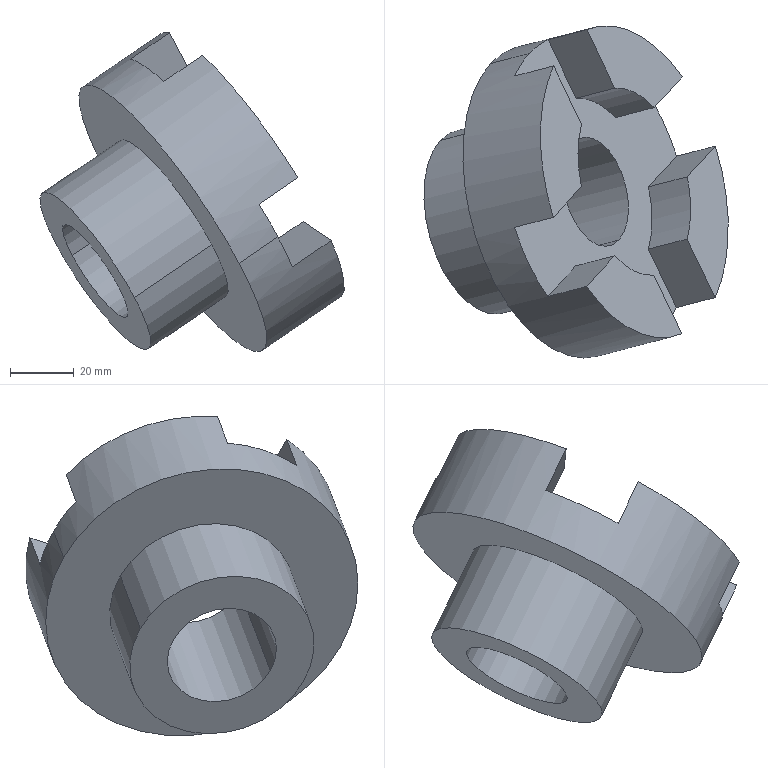Component | SolidWorks | CrusherFrameCoupling-1 | 1 solid | 25 faces | box 95.28 x 104.07 x 100.03 mm | volume 201382 mm3 | plane 15 | cylinder 10 | commonest cylinder face diameters 60 x4 59 x2 100 x2 35 x2
STEP:
#1=COLOUR_RGB('',0.7922,0.8196,0.9333);
#2=FILL_AREA_STYLE_COLOUR('',#1);
#3=FILL_AREA_STYLE('',(#2));
#4=SURFACE_STYLE_FILL_AREA(#3);
#5=SURFACE_SIDE_STYLE('',(#4));
#6=SURFACE_STYLE_USAGE(.BOTH.,#5);
#7=PRESENTATION_STYLE_ASSIGNMENT((#6));
#8=CARTESIAN_POINT('',(13.885,-5.17,1.625));
#9=VERTEX_POINT('',#8);
#10=CARTESIAN_POINT('',(14.849,-7.18,0.9731));
#11=VERTEX_POINT('',#10);
#12=CARTESIAN_POINT('',(14.367,-6.175,1.299));
#13=DIRECTION('',(0.8088,0.2094,0.5495));
#14=DIRECTION('',(-0.4148,0.8655,0.2808));
#15=AXIS2_PLACEMENT_3D('',#12,#13,#14);
#16=CIRCLE('',#15,1.161);
#17=EDGE_CURVE('',#9,#11,#16,.T.);
#18=ORIENTED_EDGE('',*,*,#17,.T.);
#19=CARTESIAN_POINT('',(15.804,-6.933,1.622));
#20=VERTEX_POINT('',#19);
#21=CARTESIAN_POINT('',(16.76,-6.685,2.271));
#22=DIRECTION('',(0.8088,0.2094,0.5495));
#23=VECTOR('',#22,39.37);
#24=LINE('',#21,#23);
#25=EDGE_CURVE('',#11,#20,#24,.T.);
#26=ORIENTED_EDGE('',*,*,#25,.T.);
#27=CARTESIAN_POINT('',(14.841,-4.922,2.274));
#28=VERTEX_POINT('',#27);
#29=CARTESIAN_POINT('',(15.323,-5.927,1.948));
#30=DIRECTION('',(0.8088,0.2094,0.5495));
#31=DIRECTION('',(-0.4148,0.8655,0.2808));
#32=AXIS2_PLACEMENT_3D('',#29,#30,#31);
#33=CIRCLE('',#32,1.161);
#34=EDGE_CURVE('',#28,#20,#33,.T.);
#35=ORIENTED_EDGE('',*,*,#34,.F.);
#36=CARTESIAN_POINT('',(15.796,-4.675,2.923));
#37=DIRECTION('',(0.8088,0.2094,0.5495));
#38=VECTOR('',#37,39.37);
#39=LINE('',#36,#38);
#40=EDGE_CURVE('',#9,#28,#39,.T.);
#41=ORIENTED_EDGE('',*,*,#40,.F.);
#42=EDGE_LOOP('',(#18,#26,#35,#41));
#43=FACE_OUTER_BOUND('',#42,.T.);
#44=CARTESIAN_POINT('',(16.278,-5.68,2.597));
#45=DIRECTION('',(0.8088,0.2094,0.5495));
#46=DIRECTION('',(-0.4148,0.8655,0.2808));
#47=AXIS2_PLACEMENT_3D('',#44,#45,#46);
#48=CYLINDRICAL_SURFACE('',#47,1.161);
#49=ADVANCED_FACE('',(#43),#48,.T.);
#50=CARTESIAN_POINT('',(14.506,-4.224,2.501));
#51=VERTEX_POINT('',#50);
#52=CARTESIAN_POINT('',(16.139,-7.631,1.395));
#53=VERTEX_POINT('',#52);
#54=CARTESIAN_POINT('',(15.323,-5.927,1.948));
#55=DIRECTION('',(0.8088,0.2094,0.5495));
#56=DIRECTION('',(-0.4148,0.8655,0.2808));
#57=AXIS2_PLACEMENT_3D('',#54,#55,#56);
#58=CIRCLE('',#57,1.969);
#59=EDGE_CURVE('',#51,#53,#58,.T.);
#60=ORIENTED_EDGE('',*,*,#59,.T.);
#61=CARTESIAN_POINT('',(16.617,-7.507,1.72));
#62=VERTEX_POINT('',#61);
#63=CARTESIAN_POINT('',(17.095,-7.384,2.044));
#64=DIRECTION('',(0.8088,0.2094,0.5495));
#65=VECTOR('',#64,39.37);
#66=LINE('',#63,#65);
#67=EDGE_CURVE('',#53,#62,#66,.T.);
#68=ORIENTED_EDGE('',*,*,#67,.T.);
#69=CARTESIAN_POINT('',(16.386,-7.677,2.125));
#70=VERTEX_POINT('',#69);
#71=CARTESIAN_POINT('',(15.8,-5.804,2.273));
#72=DIRECTION('',(-0.8088,-0.2094,-0.5495));
#73=DIRECTION('',(-0.4168,-0.4551,0.7869));
#74=AXIS2_PLACEMENT_3D('',#71,#72,#73);
#75=CIRCLE('',#74,1.969);
#76=EDGE_CURVE('',#62,#70,#75,.T.);
#77=ORIENTED_EDGE('',*,*,#76,.T.);
#78=CARTESIAN_POINT('',(16.864,-7.554,2.449));
#79=VERTEX_POINT('',#78);
#80=CARTESIAN_POINT('',(16.864,-7.554,2.449));
#81=DIRECTION('',(0.8088,0.2094,0.5495));
#82=VECTOR('',#81,39.37);
#83=LINE('',#80,#82);
#84=EDGE_CURVE('',#70,#79,#83,.T.);
#85=ORIENTED_EDGE('',*,*,#84,.T.);
#86=CARTESIAN_POINT('',(15.688,-6.973,3.959));
#87=VERTEX_POINT('',#86);
#88=CARTESIAN_POINT('',(16.278,-5.68,2.597));
#89=DIRECTION('',(0.8088,0.2094,0.5495));
#90=DIRECTION('',(-0.4148,0.8655,0.2808));
#91=AXIS2_PLACEMENT_3D('',#88,#89,#90);
#92=CIRCLE('',#91,1.969);
#93=EDGE_CURVE('',#87,#79,#92,.T.);
#94=ORIENTED_EDGE('',*,*,#93,.F.);
#95=CARTESIAN_POINT('',(15.21,-7.097,3.634));
#96=VERTEX_POINT('',#95);
#97=CARTESIAN_POINT('',(15.688,-6.973,3.959));
#98=DIRECTION('',(-0.8088,-0.2094,-0.5495));
#99=VECTOR('',#98,39.37);
#100=LINE('',#97,#99);
#101=EDGE_CURVE('',#87,#96,#100,.T.);
#102=ORIENTED_EDGE('',*,*,#101,.T.);
#103=CARTESIAN_POINT('',(14.802,-6.245,3.911));
#104=VERTEX_POINT('',#103);
#105=CARTESIAN_POINT('',(15.8,-5.804,2.273));
#106=DIRECTION('',(-0.8088,-0.2094,-0.5495));
#107=DIRECTION('',(0.4148,-0.8655,-0.2808));
#108=AXIS2_PLACEMENT_3D('',#105,#106,#107);
#109=CIRCLE('',#108,1.969);
#110=EDGE_CURVE('',#96,#104,#109,.T.);
#111=ORIENTED_EDGE('',*,*,#110,.T.);
#112=CARTESIAN_POINT('',(15.279,-6.122,4.235));
#113=VERTEX_POINT('',#112);
#114=CARTESIAN_POINT('',(15.279,-6.122,4.235));
#115=DIRECTION('',(0.8088,0.2094,0.5495));
#116=VECTOR('',#115,39.37);
#117=LINE('',#114,#116);
#118=EDGE_CURVE('',#104,#113,#117,.T.);
#119=ORIENTED_EDGE('',*,*,#118,.T.);
#120=CARTESIAN_POINT('',(15.282,-4.254,3.52));
#121=VERTEX_POINT('',#120);
#122=CARTESIAN_POINT('',(16.278,-5.68,2.597));
#123=DIRECTION('',(0.8088,0.2094,0.5495));
#124=DIRECTION('',(-0.4148,0.8655,0.2808));
#125=AXIS2_PLACEMENT_3D('',#122,#123,#124);
#126=CIRCLE('',#125,1.969);
#127=EDGE_CURVE('',#121,#113,#126,.T.);
#128=ORIENTED_EDGE('',*,*,#127,.F.);
#129=CARTESIAN_POINT('',(14.804,-4.378,3.195));
#130=VERTEX_POINT('',#129);
#131=CARTESIAN_POINT('',(15.282,-4.254,3.52));
#132=DIRECTION('',(-0.8088,-0.2094,-0.5495));
#133=VECTOR('',#132,39.37);
#134=LINE('',#131,#133);
#135=EDGE_CURVE('',#121,#130,#134,.T.);
#136=ORIENTED_EDGE('',*,*,#135,.T.);
#137=CARTESIAN_POINT('',(14.984,-4.1,2.825));
#138=VERTEX_POINT('',#137);
#139=CARTESIAN_POINT('',(15.8,-5.804,2.273));
#140=DIRECTION('',(-0.8088,-0.2094,-0.5495));
#141=DIRECTION('',(0.4148,-0.8655,-0.2808));
#142=AXIS2_PLACEMENT_3D('',#139,#140,#141);
#143=CIRCLE('',#142,1.969);
#144=EDGE_CURVE('',#130,#138,#143,.T.);
#145=ORIENTED_EDGE('',*,*,#144,.T.);
#146=CARTESIAN_POINT('',(15.461,-3.976,3.15));
#147=DIRECTION('',(0.8088,0.2094,0.5495));
#148=VECTOR('',#147,39.37);
#149=LINE('',#146,#148);
#150=EDGE_CURVE('',#51,#138,#149,.T.);
#151=ORIENTED_EDGE('',*,*,#150,.F.);
#152=EDGE_LOOP('',(#60,#68,#77,#85,#94,#102,#111,#119,#128,#136,#145,#151));
#153=FACE_OUTER_BOUND('',#152,.T.);
#154=CARTESIAN_POINT('',(16.278,-5.68,2.597));
#155=DIRECTION('',(0.8088,0.2094,0.5495));
#156=DIRECTION('',(-0.4148,0.8655,0.2808));
#157=AXIS2_PLACEMENT_3D('',#154,#155,#156);
#158=CYLINDRICAL_SURFACE('',#157,1.969);
#159=ADVANCED_FACE('',(#153),#158,.T.);
#160=CARTESIAN_POINT('',(14.653,-6.771,1.106));
#161=VERTEX_POINT('',#160);
#162=CARTESIAN_POINT('',(14.081,-5.579,1.493));
#163=VERTEX_POINT('',#162);
#164=CARTESIAN_POINT('',(14.367,-6.175,1.299));
#165=DIRECTION('',(0.8088,0.2094,0.5495));
#166=DIRECTION('',(-0.4148,0.8655,0.2808));
#167=AXIS2_PLACEMENT_3D('',#164,#165,#166);
#168=CIRCLE('',#167,0.689);
#169=EDGE_CURVE('',#161,#163,#168,.T.);
#170=ORIENTED_EDGE('',*,*,#169,.F.);
#171=CARTESIAN_POINT('',(16.086,-6.4,2.079));
#172=VERTEX_POINT('',#171);
#173=CARTESIAN_POINT('',(16.564,-6.276,2.404));
#174=DIRECTION('',(0.8088,0.2094,0.5495));
#175=VECTOR('',#174,39.37);
#176=LINE('',#173,#175);
#177=EDGE_CURVE('',#161,#172,#176,.T.);
#178=ORIENTED_EDGE('',*,*,#177,.T.);
#179=CARTESIAN_POINT('',(15.514,-5.207,2.466));
#180=VERTEX_POINT('',#179);
#181=CARTESIAN_POINT('',(15.8,-5.804,2.273));
#182=DIRECTION('',(0.8088,0.2094,0.5495));
#183=DIRECTION('',(-0.4168,-0.4551,0.7869));
#184=AXIS2_PLACEMENT_3D('',#181,#182,#183);
#185=CIRCLE('',#184,0.689);
#186=EDGE_CURVE('',#172,#180,#185,.T.);
#187=ORIENTED_EDGE('',*,*,#186,.T.);
#188=CARTESIAN_POINT('',(15.992,-5.084,2.791));
#189=DIRECTION('',(0.8088,0.2094,0.5495));
#190=VECTOR('',#189,39.37);
#191=LINE('',#188,#190);
#192=EDGE_CURVE('',#163,#180,#191,.T.);
#193=ORIENTED_EDGE('',*,*,#192,.F.);
#194=EDGE_LOOP('',(#170,#178,#187,#193));
#195=FACE_OUTER_BOUND('',#194,.T.);
#196=CARTESIAN_POINT('',(16.278,-5.68,2.597));
#197=DIRECTION('',(0.8088,0.2094,0.5495));
#198=DIRECTION('',(-0.4148,0.8655,0.2808));
#199=AXIS2_PLACEMENT_3D('',#196,#197,#198);
#200=CYLINDRICAL_SURFACE('',#199,0.689);
#201=ADVANCED_FACE('',(#195),#200,.F.);
#202=CARTESIAN_POINT('',(16.93,-5.617,1.614));
#203=VERTEX_POINT('',#202);
#204=CARTESIAN_POINT('',(17.276,-5.239,0.9592));
#205=VERTEX_POINT('',#204);
#206=CARTESIAN_POINT('',(15.662,-7.002,4.008));
#207=DIRECTION('',(0.4168,0.4551,-0.7869));
#208=VECTOR('',#207,39.37);
#209=LINE('',#206,#208);
#210=EDGE_CURVE('',#203,#205,#209,.T.);
#211=ORIENTED_EDGE('',*,*,#210,.F.);
#212=CARTESIAN_POINT('',(16.928,-6.385,1.908));
#213=VERTEX_POINT('',#212);
#214=CARTESIAN_POINT('',(16.278,-5.68,2.597));
#215=DIRECTION('',(0.8088,0.2094,0.5495));
#216=DIRECTION('',(-0.4148,0.8655,0.2808));
#217=AXIS2_PLACEMENT_3D('',#214,#215,#216);
#218=CIRCLE('',#217,1.181);
#219=EDGE_CURVE('',#213,#203,#218,.T.);
#220=ORIENTED_EDGE('',*,*,#219,.F.);
#221=CARTESIAN_POINT('',(17.274,-7.106,1.675));
#222=VERTEX_POINT('',#221);
#223=CARTESIAN_POINT('',(17.3,-7.16,1.657));
#224=DIRECTION('',(-0.4148,0.8655,0.2808));
#225=VECTOR('',#224,39.37);
#226=LINE('',#223,#225);
#227=EDGE_CURVE('',#222,#213,#226,.T.);
#228=ORIENTED_EDGE('',*,*,#227,.F.);
#229=CARTESIAN_POINT('',(16.278,-5.68,2.597));
#230=DIRECTION('',(0.8088,0.2094,0.5495));
#231=DIRECTION('',(-0.4148,0.8655,0.2808));
#232=AXIS2_PLACEMENT_3D('',#229,#230,#231);
#233=CIRCLE('',#232,1.969);
#234=EDGE_CURVE('',#222,#205,#233,.T.);
#235=ORIENTED_EDGE('',*,*,#234,.T.);
#236=EDGE_LOOP('',(#211,#220,#228,#235));
#237=FACE_OUTER_BOUND('',#236,.T.);
#238=CARTESIAN_POINT('',(15.991,-5.994,3.139));
#239=DIRECTION('',(-0.8088,-0.2094,-0.5495));
#240=DIRECTION('',(0.4148,-0.8655,-0.2808));
#241=AXIS2_PLACEMENT_3D('',#238,#239,#240);
#242=PLANE('',#241);
#243=ADVANCED_FACE('',(#237),#242,.F.);
#244=CARTESIAN_POINT('',(16.518,-6.833,2.683));
#245=VERTEX_POINT('',#244);
#246=CARTESIAN_POINT('',(16.889,-7.608,2.432));
#247=DIRECTION('',(-0.4148,0.8655,0.2808));
#248=VECTOR('',#247,39.37);
#249=LINE('',#246,#248);
#250=EDGE_CURVE('',#79,#245,#249,.T.);
#251=ORIENTED_EDGE('',*,*,#250,.T.);
#252=CARTESIAN_POINT('',(16.035,-6.595,3.304));
#253=VERTEX_POINT('',#252);
#254=CARTESIAN_POINT('',(16.278,-5.68,2.597));
#255=DIRECTION('',(0.8088,0.2094,0.5495));
#256=DIRECTION('',(-0.4148,0.8655,0.2808));
#257=AXIS2_PLACEMENT_3D('',#254,#255,#256);
#258=CIRCLE('',#257,1.181);
#259=EDGE_CURVE('',#253,#245,#258,.T.);
#260=ORIENTED_EDGE('',*,*,#259,.F.);
#261=CARTESIAN_POINT('',(15.662,-7.002,4.008));
#262=DIRECTION('',(0.4168,0.4551,-0.7869));
#263=VECTOR('',#262,39.37);
#264=LINE('',#261,#263);
#265=EDGE_CURVE('',#87,#253,#264,.T.);
#266=ORIENTED_EDGE('',*,*,#265,.F.);
#267=ORIENTED_EDGE('',*,*,#93,.T.);
#268=EDGE_LOOP('',(#251,#260,#266,#267));
#269=FACE_OUTER_BOUND('',#268,.T.);
#270=CARTESIAN_POINT('',(15.991,-5.994,3.139));
#271=DIRECTION('',(-0.8088,-0.2094,-0.5495));
#272=DIRECTION('',(0.4148,-0.8655,-0.2808));
#273=AXIS2_PLACEMENT_3D('',#270,#271,#272);
#274=PLANE('',#273);
#275=ADVANCED_FACE('',(#269),#274,.F.);
#276=CARTESIAN_POINT('',(15.626,-5.743,3.58));
#277=VERTEX_POINT('',#276);
#278=CARTESIAN_POINT('',(15.253,-6.15,4.284));
#279=DIRECTION('',(0.4168,0.4551,-0.7869));
#280=VECTOR('',#279,39.37);
#281=LINE('',#278,#280);
#282=EDGE_CURVE('',#113,#277,#281,.T.);
#283=ORIENTED_EDGE('',*,*,#282,.T.);
#284=CARTESIAN_POINT('',(15.627,-4.975,3.286));
#285=VERTEX_POINT('',#284);
#286=CARTESIAN_POINT('',(16.278,-5.68,2.597));
#287=DIRECTION('',(0.8088,0.2094,0.5495));
#288=DIRECTION('',(-0.4148,0.8655,0.2808));
#289=AXIS2_PLACEMENT_3D('',#286,#287,#288);
#290=CIRCLE('',#289,1.181);
#291=EDGE_CURVE('',#285,#277,#290,.T.);
#292=ORIENTED_EDGE('',*,*,#291,.F.);
#293=CARTESIAN_POINT('',(15.256,-4.2,3.537));
#294=DIRECTION('',(0.4148,-0.8655,-0.2808));
#295=VECTOR('',#294,39.37);
#296=LINE('',#293,#295);
#297=EDGE_CURVE('',#121,#285,#296,.T.);
#298=ORIENTED_EDGE('',*,*,#297,.F.);
#299=ORIENTED_EDGE('',*,*,#127,.T.);
#300=EDGE_LOOP('',(#283,#292,#298,#299));
#301=FACE_OUTER_BOUND('',#300,.T.);
#302=CARTESIAN_POINT('',(15.991,-5.994,3.139));
#303=DIRECTION('',(-0.8088,-0.2094,-0.5495));
#304=DIRECTION('',(0.4148,-0.8655,-0.2808));
#305=AXIS2_PLACEMENT_3D('',#302,#303,#304);
#306=PLANE('',#305);
#307=ADVANCED_FACE('',(#301),#306,.F.);
#308=ORIENTED_EDGE('',*,*,#177,.F.);
#309=CARTESIAN_POINT('',(14.367,-6.175,1.299));
#310=DIRECTION('',(0.8088,0.2094,0.5495));
#311=DIRECTION('',(-0.4148,0.8655,0.2808));
#312=AXIS2_PLACEMENT_3D('',#309,#310,#311);
#313=CIRCLE('',#312,0.689);
#314=EDGE_CURVE('',#163,#161,#313,.T.);
#315=ORIENTED_EDGE('',*,*,#314,.F.);
#316=ORIENTED_EDGE('',*,*,#192,.T.);
#317=CARTESIAN_POINT('',(15.8,-5.804,2.273));
#318=DIRECTION('',(0.8088,0.2094,0.5495));
#319=DIRECTION('',(-0.4168,-0.4551,0.7869));
#320=AXIS2_PLACEMENT_3D('',#317,#318,#319);
#321=CIRCLE('',#320,0.689);
#322=EDGE_CURVE('',#180,#172,#321,.T.);
#323=ORIENTED_EDGE('',*,*,#322,.T.);
#324=EDGE_LOOP('',(#308,#315,#316,#323));
#325=FACE_OUTER_BOUND('',#324,.T.);
#326=CARTESIAN_POINT('',(16.278,-5.68,2.597));
#327=DIRECTION('',(0.8088,0.2094,0.5495));
#328=DIRECTION('',(-0.4148,0.8655,0.2808));
#329=AXIS2_PLACEMENT_3D('',#326,#327,#328);
#330=CYLINDRICAL_SURFACE('',#329,0.689);
#331=ADVANCED_FACE('',(#325),#330,.F.);
#332=CARTESIAN_POINT('',(15.692,-3.807,2.745));
#333=VERTEX_POINT('',#332);
#334=CARTESIAN_POINT('',(16.038,-4.527,2.511));
#335=VERTEX_POINT('',#334);
#336=CARTESIAN_POINT('',(15.666,-3.752,2.763));
#337=DIRECTION('',(0.4148,-0.8655,-0.2808));
#338=VECTOR('',#337,39.37);
#339=LINE('',#336,#338);
#340=EDGE_CURVE('',#333,#335,#339,.T.);
#341=ORIENTED_EDGE('',*,*,#340,.T.);
#342=CARTESIAN_POINT('',(16.521,-4.766,1.891));
#343=VERTEX_POINT('',#342);
#344=CARTESIAN_POINT('',(16.278,-5.68,2.597));
#345=DIRECTION('',(0.8088,0.2094,0.5495));
#346=DIRECTION('',(-0.4148,0.8655,0.2808));
#347=AXIS2_PLACEMENT_3D('',#344,#345,#346);
#348=CIRCLE('',#347,1.181);
#349=EDGE_CURVE('',#343,#335,#348,.T.);
#350=ORIENTED_EDGE('',*,*,#349,.F.);
#351=CARTESIAN_POINT('',(16.868,-4.387,1.236));
#352=VERTEX_POINT('',#351);
#353=CARTESIAN_POINT('',(16.894,-4.358,1.186));
#354=DIRECTION('',(-0.4168,-0.4551,0.7869));
#355=VECTOR('',#354,39.37);
#356=LINE('',#353,#355);
#357=EDGE_CURVE('',#352,#343,#356,.T.);
#358=ORIENTED_EDGE('',*,*,#357,.F.);
#359=CARTESIAN_POINT('',(16.278,-5.68,2.597));
#360=DIRECTION('',(0.8088,0.2094,0.5495));
#361=DIRECTION('',(-0.4148,0.8655,0.2808));
#362=AXIS2_PLACEMENT_3D('',#359,#360,#361);
#363=CIRCLE('',#362,1.969);
#364=EDGE_CURVE('',#352,#333,#363,.T.);
#365=ORIENTED_EDGE('',*,*,#364,.T.);
#366=EDGE_LOOP('',(#341,#350,#358,#365));
#367=FACE_OUTER_BOUND('',#366,.T.);
#368=CARTESIAN_POINT('',(15.991,-5.994,3.139));
#369=DIRECTION('',(-0.8088,-0.2094,-0.5495));
#370=DIRECTION('',(0.4148,-0.8655,-0.2808));
#371=AXIS2_PLACEMENT_3D('',#368,#369,#370);
#372=PLANE('',#371);
#373=ADVANCED_FACE('',(#367),#372,.F.);
#374=ORIENTED_EDGE('',*,*,#67,.F.);
#375=CARTESIAN_POINT('',(15.323,-5.927,1.948));
#376=DIRECTION('',(0.8088,0.2094,0.5495));
#377=DIRECTION('',(-0.4148,0.8655,0.2808));
#378=AXIS2_PLACEMENT_3D('',#375,#376,#377);
#379=CIRCLE('',#378,1.969);
#380=EDGE_CURVE('',#53,#51,#379,.T.);
#381=ORIENTED_EDGE('',*,*,#380,.T.);
#382=ORIENTED_EDGE('',*,*,#150,.T.);
#383=CARTESIAN_POINT('',(15.215,-3.93,2.421));
#384=VERTEX_POINT('',#383);
#385=CARTESIAN_POINT('',(15.8,-5.804,2.273));
#386=DIRECTION('',(-0.8088,-0.2094,-0.5495));
#387=DIRECTION('',(0.4148,-0.8655,-0.2808));
#388=AXIS2_PLACEMENT_3D('',#385,#386,#387);
#389=CIRCLE('',#388,1.969);
#390=EDGE_CURVE('',#138,#384,#389,.T.);
#391=ORIENTED_EDGE('',*,*,#390,.T.);
#392=CARTESIAN_POINT('',(15.692,-3.807,2.745));
#393=DIRECTION('',(0.8088,0.2094,0.5495));
#394=VECTOR('',#393,39.37);
#395=LINE('',#392,#394);
#396=EDGE_CURVE('',#384,#333,#395,.T.);
#397=ORIENTED_EDGE('',*,*,#396,.T.);
#398=ORIENTED_EDGE('',*,*,#364,.F.);
#399=CARTESIAN_POINT('',(16.39,-4.51,0.9111));
#400=VERTEX_POINT('',#399);
#401=CARTESIAN_POINT('',(16.868,-4.387,1.236));
#402=DIRECTION('',(-0.8088,-0.2094,-0.5495));
#403=VECTOR('',#402,39.37);
#404=LINE('',#401,#403);
#405=EDGE_CURVE('',#352,#400,#404,.T.);
#406=ORIENTED_EDGE('',*,*,#405,.T.);
#407=CARTESIAN_POINT('',(16.799,-5.362,0.6347));
#408=VERTEX_POINT('',#407);
#409=CARTESIAN_POINT('',(15.8,-5.804,2.273));
#410=DIRECTION('',(-0.8088,-0.2094,-0.5495));
#411=DIRECTION('',(0.4148,-0.8655,-0.2808));
#412=AXIS2_PLACEMENT_3D('',#409,#410,#411);
#413=CIRCLE('',#412,1.969);
#414=EDGE_CURVE('',#400,#408,#413,.T.);
#415=ORIENTED_EDGE('',*,*,#414,.T.);
#416=CARTESIAN_POINT('',(17.276,-5.239,0.9592));
#417=DIRECTION('',(0.8088,0.2094,0.5495));
#418=VECTOR('',#417,39.37);
#419=LINE('',#416,#418);
#420=EDGE_CURVE('',#408,#205,#419,.T.);
#421=ORIENTED_EDGE('',*,*,#420,.T.);
#422=ORIENTED_EDGE('',*,*,#234,.F.);
#423=CARTESIAN_POINT('',(16.796,-7.229,1.35));
#424=VERTEX_POINT('',#423);
#425=CARTESIAN_POINT('',(17.274,-7.106,1.675));
#426=DIRECTION('',(-0.8088,-0.2094,-0.5495));
#427=VECTOR('',#426,39.37);
#428=LINE('',#425,#427);
#429=EDGE_CURVE('',#222,#424,#428,.T.);
#430=ORIENTED_EDGE('',*,*,#429,.T.);
#431=CARTESIAN_POINT('',(15.8,-5.804,2.273));
#432=DIRECTION('',(-0.8088,-0.2094,-0.5495));
#433=DIRECTION('',(-0.4168,-0.4551,0.7869));
#434=AXIS2_PLACEMENT_3D('',#431,#432,#433);
#435=CIRCLE('',#434,1.969);
#436=EDGE_CURVE('',#424,#62,#435,.T.);
#437=ORIENTED_EDGE('',*,*,#436,.T.);
#438=EDGE_LOOP('',(#374,#381,#382,#391,#397,#398,#406,#415,#421,#422,#430,#437));
#439=FACE_OUTER_BOUND('',#438,.T.);
#440=CARTESIAN_POINT('',(16.278,-5.68,2.597));
#441=DIRECTION('',(0.8088,0.2094,0.5495));
#442=DIRECTION('',(-0.4148,0.8655,0.2808));
#443=AXIS2_PLACEMENT_3D('',#440,#441,#442);
#444=CYLINDRICAL_SURFACE('',#443,1.969);
#445=ADVANCED_FACE('',(#439),#444,.T.);
#446=ORIENTED_EDGE('',*,*,#59,.F.);
#447=ORIENTED_EDGE('',*,*,#380,.F.);
#448=EDGE_LOOP('',(#446,#447));
#449=FACE_OUTER_BOUND('',#448,.T.);
#450=ORIENTED_EDGE('',*,*,#34,.T.);
#451=CARTESIAN_POINT('',(15.323,-5.927,1.948));
#452=DIRECTION('',(0.8088,0.2094,0.5495));
#453=DIRECTION('',(-0.4148,0.8655,0.2808));
#454=AXIS2_PLACEMENT_3D('',#451,#452,#453);
#455=CIRCLE('',#454,1.161);
#456=EDGE_CURVE('',#20,#28,#455,.T.);
#457=ORIENTED_EDGE('',*,*,#456,.T.);
#458=EDGE_LOOP('',(#450,#457));
#459=FACE_BOUND('',#458,.T.);
#460=CARTESIAN_POINT('',(14.502,-6.823,3.497));
#461=DIRECTION('',(0.8088,0.2094,0.5495));
#462=DIRECTION('',(-0.4148,0.8655,0.2808));
#463=AXIS2_PLACEMENT_3D('',#460,#461,#462);
#464=PLANE('',#463);
#465=ADVANCED_FACE('',(#449,#459),#464,.F.);
#466=ORIENTED_EDGE('',*,*,#25,.F.);
#467=CARTESIAN_POINT('',(14.367,-6.175,1.299));
#468=DIRECTION('',(0.8088,0.2094,0.5495));
#469=DIRECTION('',(-0.4148,0.8655,0.2808));
#470=AXIS2_PLACEMENT_3D('',#467,#468,#469);
#471=CIRCLE('',#470,1.161);
#472=EDGE_CURVE('',#11,#9,#471,.T.);
#473=ORIENTED_EDGE('',*,*,#472,.T.);
#474=ORIENTED_EDGE('',*,*,#40,.T.);
#475=ORIENTED_EDGE('',*,*,#456,.F.);
#476=EDGE_LOOP('',(#466,#473,#474,#475));
#477=FACE_OUTER_BOUND('',#476,.T.);
#478=CARTESIAN_POINT('',(16.278,-5.68,2.597));
#479=DIRECTION('',(0.8088,0.2094,0.5495));
#480=DIRECTION('',(-0.4148,0.8655,0.2808));
#481=AXIS2_PLACEMENT_3D('',#478,#479,#480);
#482=CYLINDRICAL_SURFACE('',#481,1.161);
#483=ADVANCED_FACE('',(#477),#482,.T.);
#484=ORIENTED_EDGE('',*,*,#17,.F.);
#485=ORIENTED_EDGE('',*,*,#472,.F.);
#486=EDGE_LOOP('',(#484,#485));
#487=FACE_OUTER_BOUND('',#486,.T.);
#488=ORIENTED_EDGE('',*,*,#314,.T.);
#489=ORIENTED_EDGE('',*,*,#169,.T.);
#490=EDGE_LOOP('',(#488,#489));
#491=FACE_BOUND('',#490,.T.);
#492=CARTESIAN_POINT('',(13.883,-6.703,2.213));
#493=DIRECTION('',(0.8088,0.2094,0.5495));
#494=DIRECTION('',(-0.4148,0.8655,0.2808));
#495=AXIS2_PLACEMENT_3D('',#492,#493,#494);
#496=PLANE('',#495);
#497=ADVANCED_FACE('',(#487,#491),#496,.F.);
#498=CARTESIAN_POINT('',(16.041,-6.957,2.358));
#499=VERTEX_POINT('',#498);
#500=CARTESIAN_POINT('',(16.412,-7.731,2.107));
#501=DIRECTION('',(-0.4148,0.8655,0.2808));
#502=VECTOR('',#501,39.37);
#503=LINE('',#500,#502);
#504=EDGE_CURVE('',#70,#499,#503,.T.);
#505=ORIENTED_EDGE('',*,*,#504,.T.);
#506=CARTESIAN_POINT('',(16.041,-6.957,2.358));
#507=DIRECTION('',(0.8088,0.2094,0.5495));
#508=VECTOR('',#507,39.37);
#509=LINE('',#506,#508);
#510=EDGE_CURVE('',#499,#245,#509,.T.);
#511=ORIENTED_EDGE('',*,*,#510,.T.);
#512=ORIENTED_EDGE('',*,*,#250,.F.);
#513=ORIENTED_EDGE('',*,*,#84,.F.);
#514=EDGE_LOOP('',(#505,#511,#512,#513));
#515=FACE_OUTER_BOUND('',#514,.T.);
#516=CARTESIAN_POINT('',(16.889,-7.608,2.432));
#517=DIRECTION('',(-0.4168,-0.4551,0.7869));
#518=DIRECTION('',(-0.4148,0.8655,0.2808));
#519=AXIS2_PLACEMENT_3D('',#516,#517,#518);
#520=PLANE('',#519);
#521=ADVANCED_FACE('',(#515),#520,.F.);
#522=CARTESIAN_POINT('',(15.557,-6.718,2.979));
#523=VERTEX_POINT('',#522);
#524=CARTESIAN_POINT('',(15.184,-7.126,3.684));
#525=DIRECTION('',(0.4168,0.4551,-0.7869));
#526=VECTOR('',#525,39.37);
#527=LINE('',#524,#526);
#528=EDGE_CURVE('',#96,#523,#527,.T.);
#529=ORIENTED_EDGE('',*,*,#528,.T.);
#530=CARTESIAN_POINT('',(15.8,-5.804,2.273));
#531=DIRECTION('',(0.8088,0.2094,0.5495));
#532=DIRECTION('',(-0.4148,0.8655,0.2808));
#533=AXIS2_PLACEMENT_3D('',#530,#531,#532);
#534=CIRCLE('',#533,1.181);
#535=EDGE_CURVE('',#523,#499,#534,.T.);
#536=ORIENTED_EDGE('',*,*,#535,.T.);
#537=ORIENTED_EDGE('',*,*,#504,.F.);
#538=ORIENTED_EDGE('',*,*,#76,.F.);
#539=ORIENTED_EDGE('',*,*,#436,.F.);
#540=CARTESIAN_POINT('',(16.451,-6.509,1.584));
#541=VERTEX_POINT('',#540);
#542=CARTESIAN_POINT('',(16.822,-7.284,1.333));
#543=DIRECTION('',(-0.4148,0.8655,0.2808));
#544=VECTOR('',#543,39.37);
#545=LINE('',#542,#544);
#546=EDGE_CURVE('',#424,#541,#545,.T.);
#547=ORIENTED_EDGE('',*,*,#546,.T.);
#548=CARTESIAN_POINT('',(16.452,-5.741,1.29));
#549=VERTEX_POINT('',#548);
#550=CARTESIAN_POINT('',(15.8,-5.804,2.273));
#551=DIRECTION('',(0.8088,0.2094,0.5495));
#552=DIRECTION('',(-0.4148,0.8655,0.2808));
#553=AXIS2_PLACEMENT_3D('',#550,#551,#552);
#554=CIRCLE('',#553,1.181);
#555=EDGE_CURVE('',#541,#549,#554,.T.);
#556=ORIENTED_EDGE('',*,*,#555,.T.);
#557=CARTESIAN_POINT('',(15.184,-7.126,3.684));
#558=DIRECTION('',(0.4168,0.4551,-0.7869));
#559=VECTOR('',#558,39.37);
#560=LINE('',#557,#559);
#561=EDGE_CURVE('',#549,#408,#560,.T.);
#562=ORIENTED_EDGE('',*,*,#561,.T.);
#563=ORIENTED_EDGE('',*,*,#414,.F.);
#564=CARTESIAN_POINT('',(16.044,-4.889,1.566));
#565=VERTEX_POINT('',#564);
#566=CARTESIAN_POINT('',(16.417,-4.482,0.8619));
#567=DIRECTION('',(-0.4168,-0.4551,0.7869));
#568=VECTOR('',#567,39.37);
#569=LINE('',#566,#568);
#570=EDGE_CURVE('',#400,#565,#569,.T.);
#571=ORIENTED_EDGE('',*,*,#570,.T.);
#572=CARTESIAN_POINT('',(15.56,-4.651,2.187));
#573=VERTEX_POINT('',#572);
#574=CARTESIAN_POINT('',(15.8,-5.804,2.273));
#575=DIRECTION('',(0.8088,0.2094,0.5495));
#576=DIRECTION('',(-0.4148,0.8655,0.2808));
#577=AXIS2_PLACEMENT_3D('',#574,#575,#576);
#578=CIRCLE('',#577,1.181);
#579=EDGE_CURVE('',#565,#573,#578,.T.);
#580=ORIENTED_EDGE('',*,*,#579,.T.);
#581=CARTESIAN_POINT('',(15.189,-3.876,2.438));
#582=DIRECTION('',(0.4148,-0.8655,-0.2808));
#583=VECTOR('',#582,39.37);
#584=LINE('',#581,#583);
#585=EDGE_CURVE('',#384,#573,#584,.T.);
#586=ORIENTED_EDGE('',*,*,#585,.F.);
#587=ORIENTED_EDGE('',*,*,#390,.F.);
#588=ORIENTED_EDGE('',*,*,#144,.F.);
#589=CARTESIAN_POINT('',(15.15,-5.098,2.961));
#590=VERTEX_POINT('',#589);
#591=CARTESIAN_POINT('',(14.779,-4.324,3.213));
#592=DIRECTION('',(0.4148,-0.8655,-0.2808));
#593=VECTOR('',#592,39.37);
#594=LINE('',#591,#593);
#595=EDGE_CURVE('',#130,#590,#594,.T.);
#596=ORIENTED_EDGE('',*,*,#595,.T.);
#597=CARTESIAN_POINT('',(15.149,-5.866,3.256));
#598=VERTEX_POINT('',#597);
#599=CARTESIAN_POINT('',(15.8,-5.804,2.273));
#600=DIRECTION('',(0.8088,0.2094,0.5495));
#601=DIRECTION('',(-0.4148,0.8655,0.2808));
#602=AXIS2_PLACEMENT_3D('',#599,#600,#601);
#603=CIRCLE('',#602,1.181);
#604=EDGE_CURVE('',#590,#598,#603,.T.);
#605=ORIENTED_EDGE('',*,*,#604,.T.);
#606=CARTESIAN_POINT('',(14.776,-6.274,3.96));
#607=DIRECTION('',(0.4168,0.4551,-0.7869));
#608=VECTOR('',#607,39.37);
#609=LINE('',#606,#608);
#610=EDGE_CURVE('',#104,#598,#609,.T.);
#611=ORIENTED_EDGE('',*,*,#610,.F.);
#612=ORIENTED_EDGE('',*,*,#110,.F.);
#613=EDGE_LOOP('',(#529,#536,#537,#538,#539,#547,#556,#562,#563,#571,#580,#586,#587,#588,#596,#605,#611,#612));
#614=FACE_OUTER_BOUND('',#613,.T.);
#615=ORIENTED_EDGE('',*,*,#322,.F.);
#616=ORIENTED_EDGE('',*,*,#186,.F.);
#617=EDGE_LOOP('',(#615,#616));
#618=FACE_BOUND('',#617,.T.);
#619=CARTESIAN_POINT('',(16.412,-7.731,2.107));
#620=DIRECTION('',(-0.8088,-0.2094,-0.5495));
#621=DIRECTION('',(-0.4168,-0.4551,0.7869));
#622=AXIS2_PLACEMENT_3D('',#619,#620,#621);
#623=PLANE('',#622);
#624=ADVANCED_FACE('',(#614,#618),#623,.F.);
#625=ORIENTED_EDGE('',*,*,#227,.T.);
#626=CARTESIAN_POINT('',(16.451,-6.509,1.584));
#627=DIRECTION('',(-0.8088,-0.2094,-0.5495));
#628=VECTOR('',#627,39.37);
#629=LINE('',#626,#628);
#630=EDGE_CURVE('',#213,#541,#629,.T.);
#631=ORIENTED_EDGE('',*,*,#630,.T.);
#632=ORIENTED_EDGE('',*,*,#546,.F.);
#633=ORIENTED_EDGE('',*,*,#429,.F.);
#634=EDGE_LOOP('',(#625,#631,#632,#633));
#635=FACE_OUTER_BOUND('',#634,.T.);
#636=CARTESIAN_POINT('',(17.3,-7.16,1.657));
#637=DIRECTION('',(0.4168,0.4551,-0.7869));
#638=DIRECTION('',(0.4148,-0.8655,-0.2808));
#639=AXIS2_PLACEMENT_3D('',#636,#637,#638);
#640=PLANE('',#639);
#641=ADVANCED_FACE('',(#635),#640,.F.);
#642=ORIENTED_EDGE('',*,*,#610,.T.);
#643=CARTESIAN_POINT('',(15.149,-5.866,3.256));
#644=DIRECTION('',(0.8088,0.2094,0.5495));
#645=VECTOR('',#644,39.37);
#646=LINE('',#643,#645);
#647=EDGE_CURVE('',#598,#277,#646,.T.);
#648=ORIENTED_EDGE('',*,*,#647,.T.);
#649=ORIENTED_EDGE('',*,*,#282,.F.);
#650=ORIENTED_EDGE('',*,*,#118,.F.);
#651=EDGE_LOOP('',(#642,#648,#649,#650));
#652=FACE_OUTER_BOUND('',#651,.T.);
#653=CARTESIAN_POINT('',(15.253,-6.15,4.284));
#654=DIRECTION('',(-0.4148,0.8655,0.2808));
#655=DIRECTION('',(0.4168,0.4551,-0.7869));
#656=AXIS2_PLACEMENT_3D('',#653,#654,#655);
#657=PLANE('',#656);
#658=ADVANCED_FACE('',(#652),#657,.F.);
#659=ORIENTED_EDGE('',*,*,#585,.T.);
#660=CARTESIAN_POINT('',(15.56,-4.651,2.187));
#661=DIRECTION('',(0.8088,0.2094,0.5495));
#662=VECTOR('',#661,39.37);
#663=LINE('',#660,#662);
#664=EDGE_CURVE('',#573,#335,#663,.T.);
#665=ORIENTED_EDGE('',*,*,#664,.T.);
#666=ORIENTED_EDGE('',*,*,#340,.F.);
#667=ORIENTED_EDGE('',*,*,#396,.F.);
#668=EDGE_LOOP('',(#659,#665,#666,#667));
#669=FACE_OUTER_BOUND('',#668,.T.);
#670=CARTESIAN_POINT('',(15.666,-3.752,2.763));
#671=DIRECTION('',(0.4168,0.4551,-0.7869));
#672=DIRECTION('',(0.4148,-0.8655,-0.2808));
#673=AXIS2_PLACEMENT_3D('',#670,#671,#672);
#674=PLANE('',#673);
#675=ADVANCED_FACE('',(#669),#674,.F.);
#676=ORIENTED_EDGE('',*,*,#297,.T.);
#677=CARTESIAN_POINT('',(15.15,-5.098,2.961));
#678=DIRECTION('',(-0.8088,-0.2094,-0.5495));
#679=VECTOR('',#678,39.37);
#680=LINE('',#677,#679);
#681=EDGE_CURVE('',#285,#590,#680,.T.);
#682=ORIENTED_EDGE('',*,*,#681,.T.);
#683=ORIENTED_EDGE('',*,*,#595,.F.);
#684=ORIENTED_EDGE('',*,*,#135,.F.);
#685=EDGE_LOOP('',(#676,#682,#683,#684));
#686=FACE_OUTER_BOUND('',#685,.T.);
#687=CARTESIAN_POINT('',(15.256,-4.2,3.537));
#688=DIRECTION('',(-0.4168,-0.4551,0.7869));
#689=DIRECTION('',(-0.4148,0.8655,0.2808));
#690=AXIS2_PLACEMENT_3D('',#687,#688,#689);
#691=PLANE('',#690);
#692=ADVANCED_FACE('',(#686),#691,.F.);
#693=ORIENTED_EDGE('',*,*,#357,.T.);
#694=CARTESIAN_POINT('',(16.044,-4.889,1.566));
#695=DIRECTION('',(-0.8088,-0.2094,-0.5495));
#696=VECTOR('',#695,39.37);
#697=LINE('',#694,#696);
#698=EDGE_CURVE('',#343,#565,#697,.T.);
#699=ORIENTED_EDGE('',*,*,#698,.T.);
#700=ORIENTED_EDGE('',*,*,#570,.F.);
#701=ORIENTED_EDGE('',*,*,#405,.F.);
#702=EDGE_LOOP('',(#693,#699,#700,#701));
#703=FACE_OUTER_BOUND('',#702,.T.);
#704=CARTESIAN_POINT('',(16.894,-4.358,1.186));
#705=DIRECTION('',(-0.4148,0.8655,0.2808));
#706=DIRECTION('',(0.4168,0.4551,-0.7869));
#707=AXIS2_PLACEMENT_3D('',#704,#705,#706);
#708=PLANE('',#707);
#709=ADVANCED_FACE('',(#703),#708,.F.);
#710=ORIENTED_EDGE('',*,*,#561,.F.);
#711=CARTESIAN_POINT('',(16.452,-5.741,1.29));
#712=DIRECTION('',(0.8088,0.2094,0.5495));
#713=VECTOR('',#712,39.37);
#714=LINE('',#711,#713);
#715=EDGE_CURVE('',#549,#203,#714,.T.);
#716=ORIENTED_EDGE('',*,*,#715,.T.);
#717=ORIENTED_EDGE('',*,*,#210,.T.);
#718=ORIENTED_EDGE('',*,*,#420,.F.);
#719=EDGE_LOOP('',(#710,#716,#717,#718));
#720=FACE_OUTER_BOUND('',#719,.T.);
#721=CARTESIAN_POINT('',(15.662,-7.002,4.008));
#722=DIRECTION('',(0.4148,-0.8655,-0.2808));
#723=DIRECTION('',(-0.4168,-0.4551,0.7869));
#724=AXIS2_PLACEMENT_3D('',#721,#722,#723);
#725=PLANE('',#724);
#726=ADVANCED_FACE('',(#720),#725,.F.);
#727=ORIENTED_EDGE('',*,*,#265,.T.);
#728=CARTESIAN_POINT('',(15.557,-6.718,2.979));
#729=DIRECTION('',(-0.8088,-0.2094,-0.5495));
#730=VECTOR('',#729,39.37);
#731=LINE('',#728,#730);
#732=EDGE_CURVE('',#253,#523,#731,.T.);
#733=ORIENTED_EDGE('',*,*,#732,.T.);
#734=ORIENTED_EDGE('',*,*,#528,.F.);
#735=ORIENTED_EDGE('',*,*,#101,.F.);
#736=EDGE_LOOP('',(#727,#733,#734,#735));
#737=FACE_OUTER_BOUND('',#736,.T.);
#738=CARTESIAN_POINT('',(15.662,-7.002,4.008));
#739=DIRECTION('',(0.4148,-0.8655,-0.2808));
#740=DIRECTION('',(-0.4168,-0.4551,0.7869));
#741=AXIS2_PLACEMENT_3D('',#738,#739,#740);
#742=PLANE('',#741);
#743=ADVANCED_FACE('',(#737),#742,.F.);
#744=ORIENTED_EDGE('',*,*,#535,.F.);
#745=ORIENTED_EDGE('',*,*,#732,.F.);
#746=ORIENTED_EDGE('',*,*,#259,.T.);
#747=ORIENTED_EDGE('',*,*,#510,.F.);
#748=EDGE_LOOP('',(#744,#745,#746,#747));
#749=FACE_OUTER_BOUND('',#748,.T.);
#750=CARTESIAN_POINT('',(15.8,-5.804,2.273));
#751=DIRECTION('',(0.8088,0.2094,0.5495));
#752=DIRECTION('',(-0.4148,0.8655,0.2808));
#753=AXIS2_PLACEMENT_3D('',#750,#751,#752);
#754=CYLINDRICAL_SURFACE('',#753,1.181);
#755=ADVANCED_FACE('',(#749),#754,.F.);
#756=ORIENTED_EDGE('',*,*,#219,.T.);
#757=ORIENTED_EDGE('',*,*,#715,.F.);
#758=ORIENTED_EDGE('',*,*,#555,.F.);
#759=ORIENTED_EDGE('',*,*,#630,.F.);
#760=EDGE_LOOP('',(#756,#757,#758,#759));
#761=FACE_OUTER_BOUND('',#760,.T.);
#762=CARTESIAN_POINT('',(15.8,-5.804,2.273));
#763=DIRECTION('',(0.8088,0.2094,0.5495));
#764=DIRECTION('',(-0.4148,0.8655,0.2808));
#765=AXIS2_PLACEMENT_3D('',#762,#763,#764);
#766=CYLINDRICAL_SURFACE('',#765,1.181);
#767=ADVANCED_FACE('',(#761),#766,.F.);
#768=ORIENTED_EDGE('',*,*,#579,.F.);
#769=ORIENTED_EDGE('',*,*,#698,.F.);
#770=ORIENTED_EDGE('',*,*,#349,.T.);
#771=ORIENTED_EDGE('',*,*,#664,.F.);
#772=EDGE_LOOP('',(#768,#769,#770,#771));
#773=FACE_OUTER_BOUND('',#772,.T.);
#774=CARTESIAN_POINT('',(15.8,-5.804,2.273));
#775=DIRECTION('',(0.8088,0.2094,0.5495));
#776=DIRECTION('',(-0.4148,0.8655,0.2808));
#777=AXIS2_PLACEMENT_3D('',#774,#775,#776);
#778=CYLINDRICAL_SURFACE('',#777,1.181);
#779=ADVANCED_FACE('',(#773),#778,.F.);
#780=ORIENTED_EDGE('',*,*,#604,.F.);
#781=ORIENTED_EDGE('',*,*,#681,.F.);
#782=ORIENTED_EDGE('',*,*,#291,.T.);
#783=ORIENTED_EDGE('',*,*,#647,.F.);
#784=EDGE_LOOP('',(#780,#781,#782,#783));
#785=FACE_OUTER_BOUND('',#784,.T.);
#786=CARTESIAN_POINT('',(15.8,-5.804,2.273));
#787=DIRECTION('',(0.8088,0.2094,0.5495));
#788=DIRECTION('',(-0.4148,0.8655,0.2808));
#789=AXIS2_PLACEMENT_3D('',#786,#787,#788);
#790=CYLINDRICAL_SURFACE('',#789,1.181);
#791=ADVANCED_FACE('',(#785),#790,.F.);
#792=CLOSED_SHELL('',(#49,#159,#201,#243,#275,#307,#331,#373,#445,#465,#483,#497,#521,#624,#641,#658,#675,#692,#709,#726,#743,#755,#767,#779,#791));
#793=MANIFOLD_SOLID_BREP('',#792);
#794=STYLED_ITEM('',(#7),#793);
#795=PRESENTATION_LAYER_ASSIGNMENT('','',(#794));
#796=CARTESIAN_POINT('',(0.,0.,0.));
#797=DIRECTION('',(0.,0.,1.));
#798=DIRECTION('',(1.,0.,0.));
#799=AXIS2_PLACEMENT_3D('',#796,#797,#798);
#800=(LENGTH_UNIT()NAMED_UNIT(*)SI_UNIT($,.METRE.));
#801=LENGTH_MEASURE_WITH_UNIT(LENGTH_MEASURE(0.0254),#800);
#802=DIMENSIONAL_EXPONENTS(1.,0.,0.,0.,0.,0.,0.);
#803=(CONVERSION_BASED_UNIT('',#801)LENGTH_UNIT()NAMED_UNIT(#802));
#804=UNCERTAINTY_MEASURE_WITH_UNIT(LENGTH_MEASURE(0.00001),#803,'','');
#805=(NAMED_UNIT(*)PLANE_ANGLE_UNIT()SI_UNIT($,.RADIAN.));
#806=(NAMED_UNIT(*)SI_UNIT($,.STERADIAN.)SOLID_ANGLE_UNIT());
#807=(GEOMETRIC_REPRESENTATION_CONTEXT(3)GLOBAL_UNCERTAINTY_ASSIGNED_CONTEXT((#804))GLOBAL_UNIT_ASSIGNED_CONTEXT((#803,#805,#806))REPRESENTATION_CONTEXT('',''));
#808=ADVANCED_BREP_SHAPE_REPRESENTATION('',(#793,#799),#807);
#809=(LENGTH_UNIT()NAMED_UNIT(*)SI_UNIT($,.METRE.));
#810=LENGTH_MEASURE_WITH_UNIT(LENGTH_MEASURE(0.0254),#809);
#811=DIMENSIONAL_EXPONENTS(1.,0.,0.,0.,0.,0.,0.);
#812=(CONVERSION_BASED_UNIT('',#810)LENGTH_UNIT()NAMED_UNIT(#811));
#813=UNCERTAINTY_MEASURE_WITH_UNIT(LENGTH_MEASURE(0.00001),#812,'','');
#814=(NAMED_UNIT(*)PLANE_ANGLE_UNIT()SI_UNIT($,.RADIAN.));
#815=(NAMED_UNIT(*)SI_UNIT($,.STERADIAN.)SOLID_ANGLE_UNIT());
#816=(GEOMETRIC_REPRESENTATION_CONTEXT(3)GLOBAL_UNCERTAINTY_ASSIGNED_CONTEXT((#813))GLOBAL_UNIT_ASSIGNED_CONTEXT((#812,#814,#815))REPRESENTATION_CONTEXT('',''));
#817=MECHANICAL_DESIGN_GEOMETRIC_PRESENTATION_REPRESENTATION('',(#794),#816);